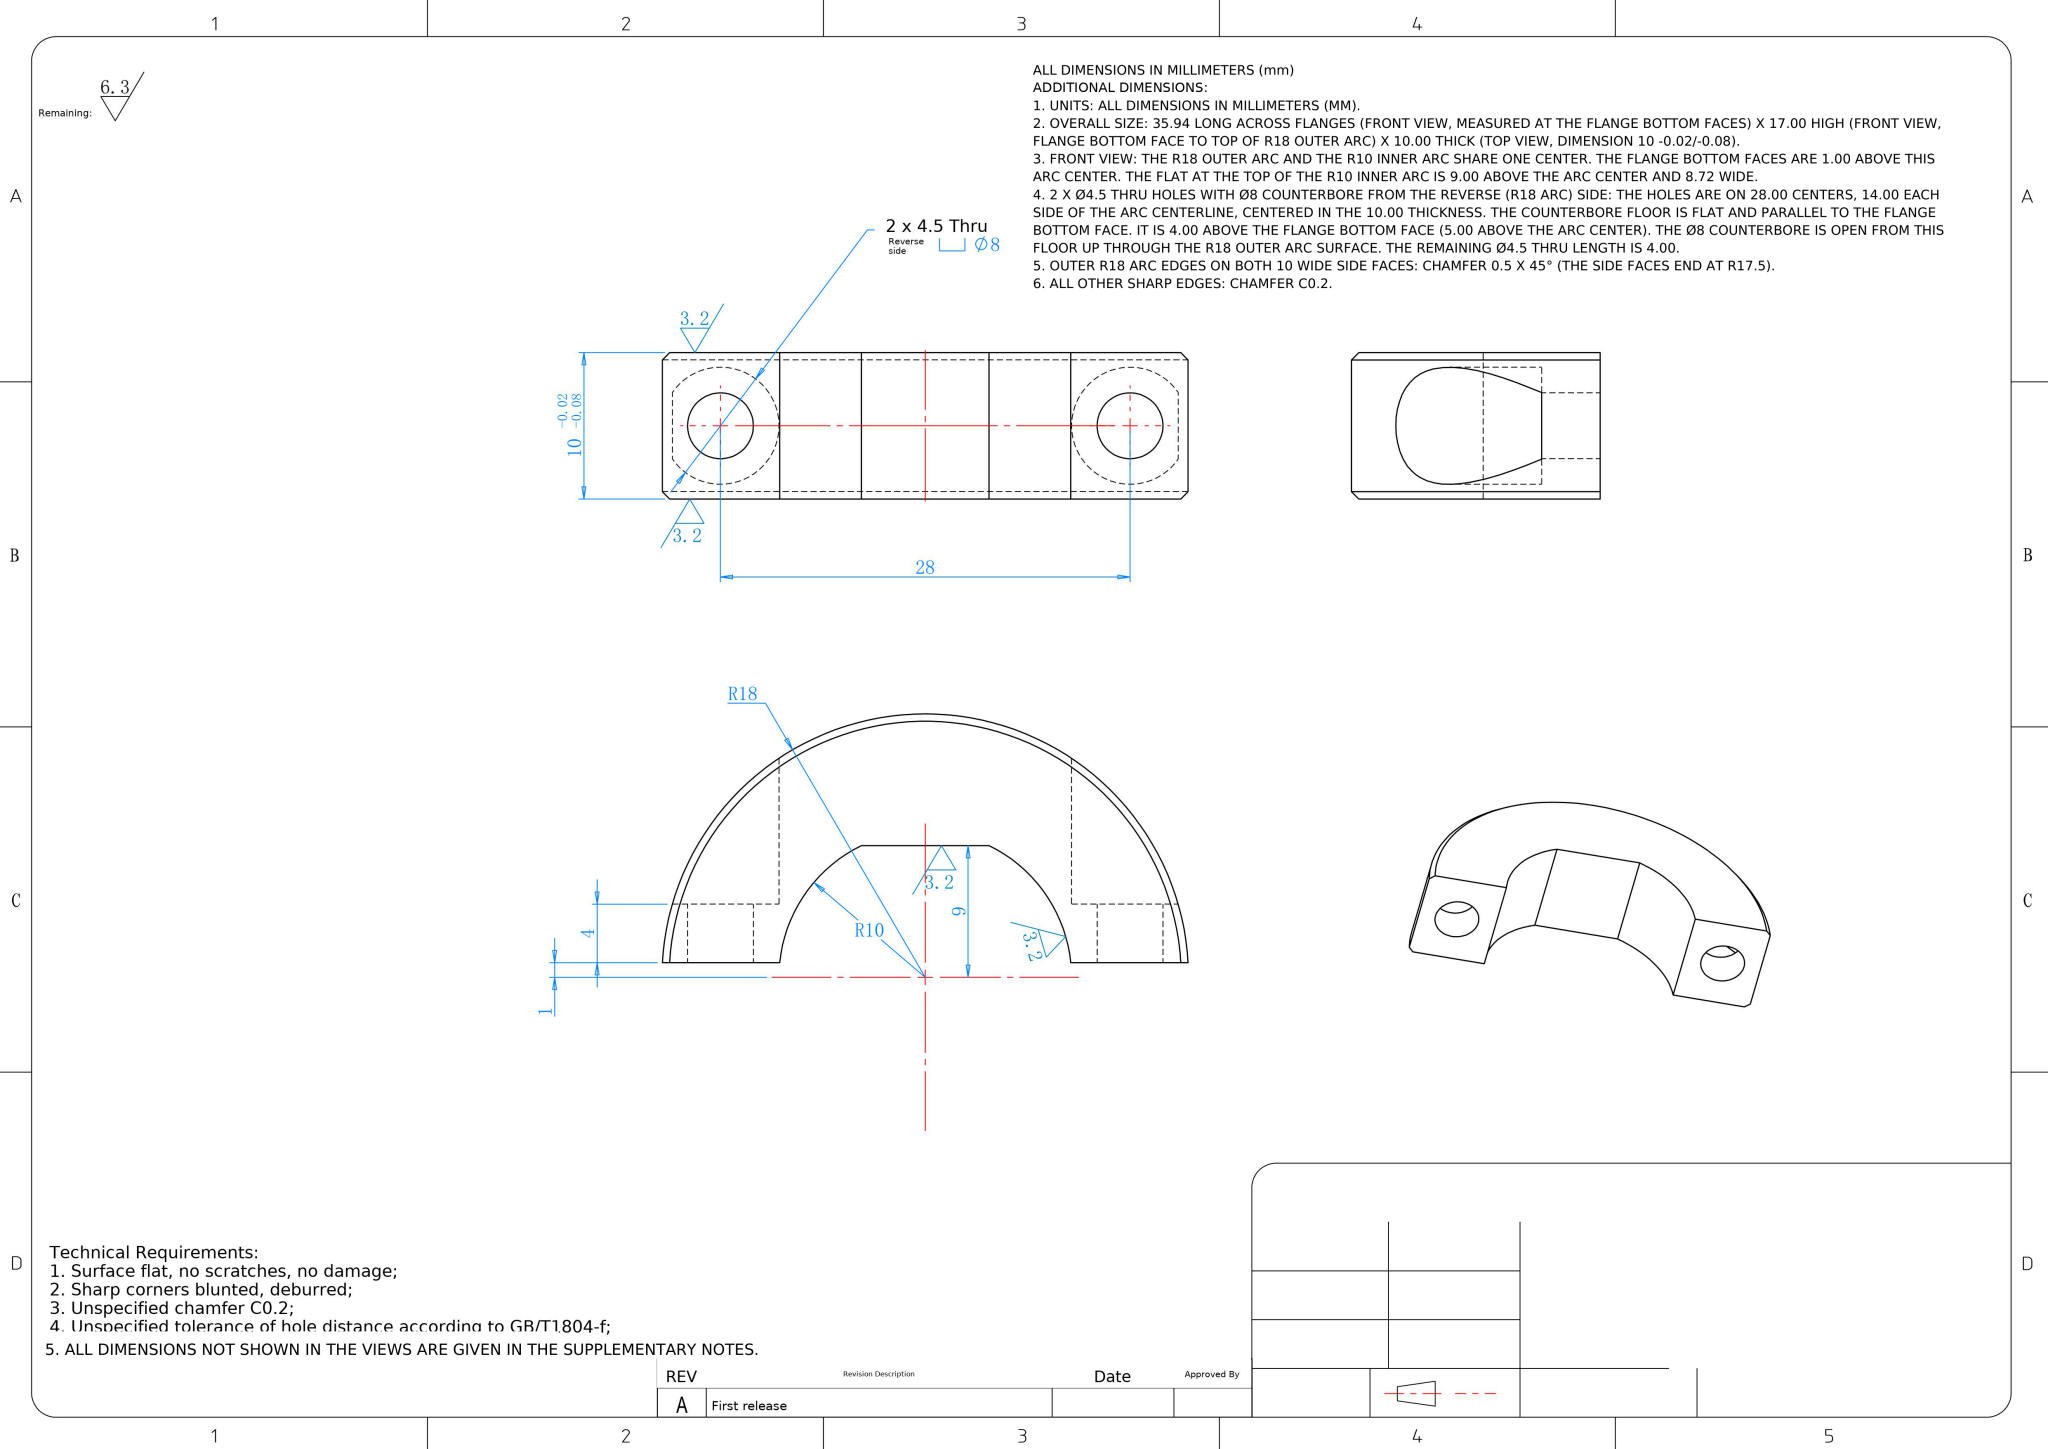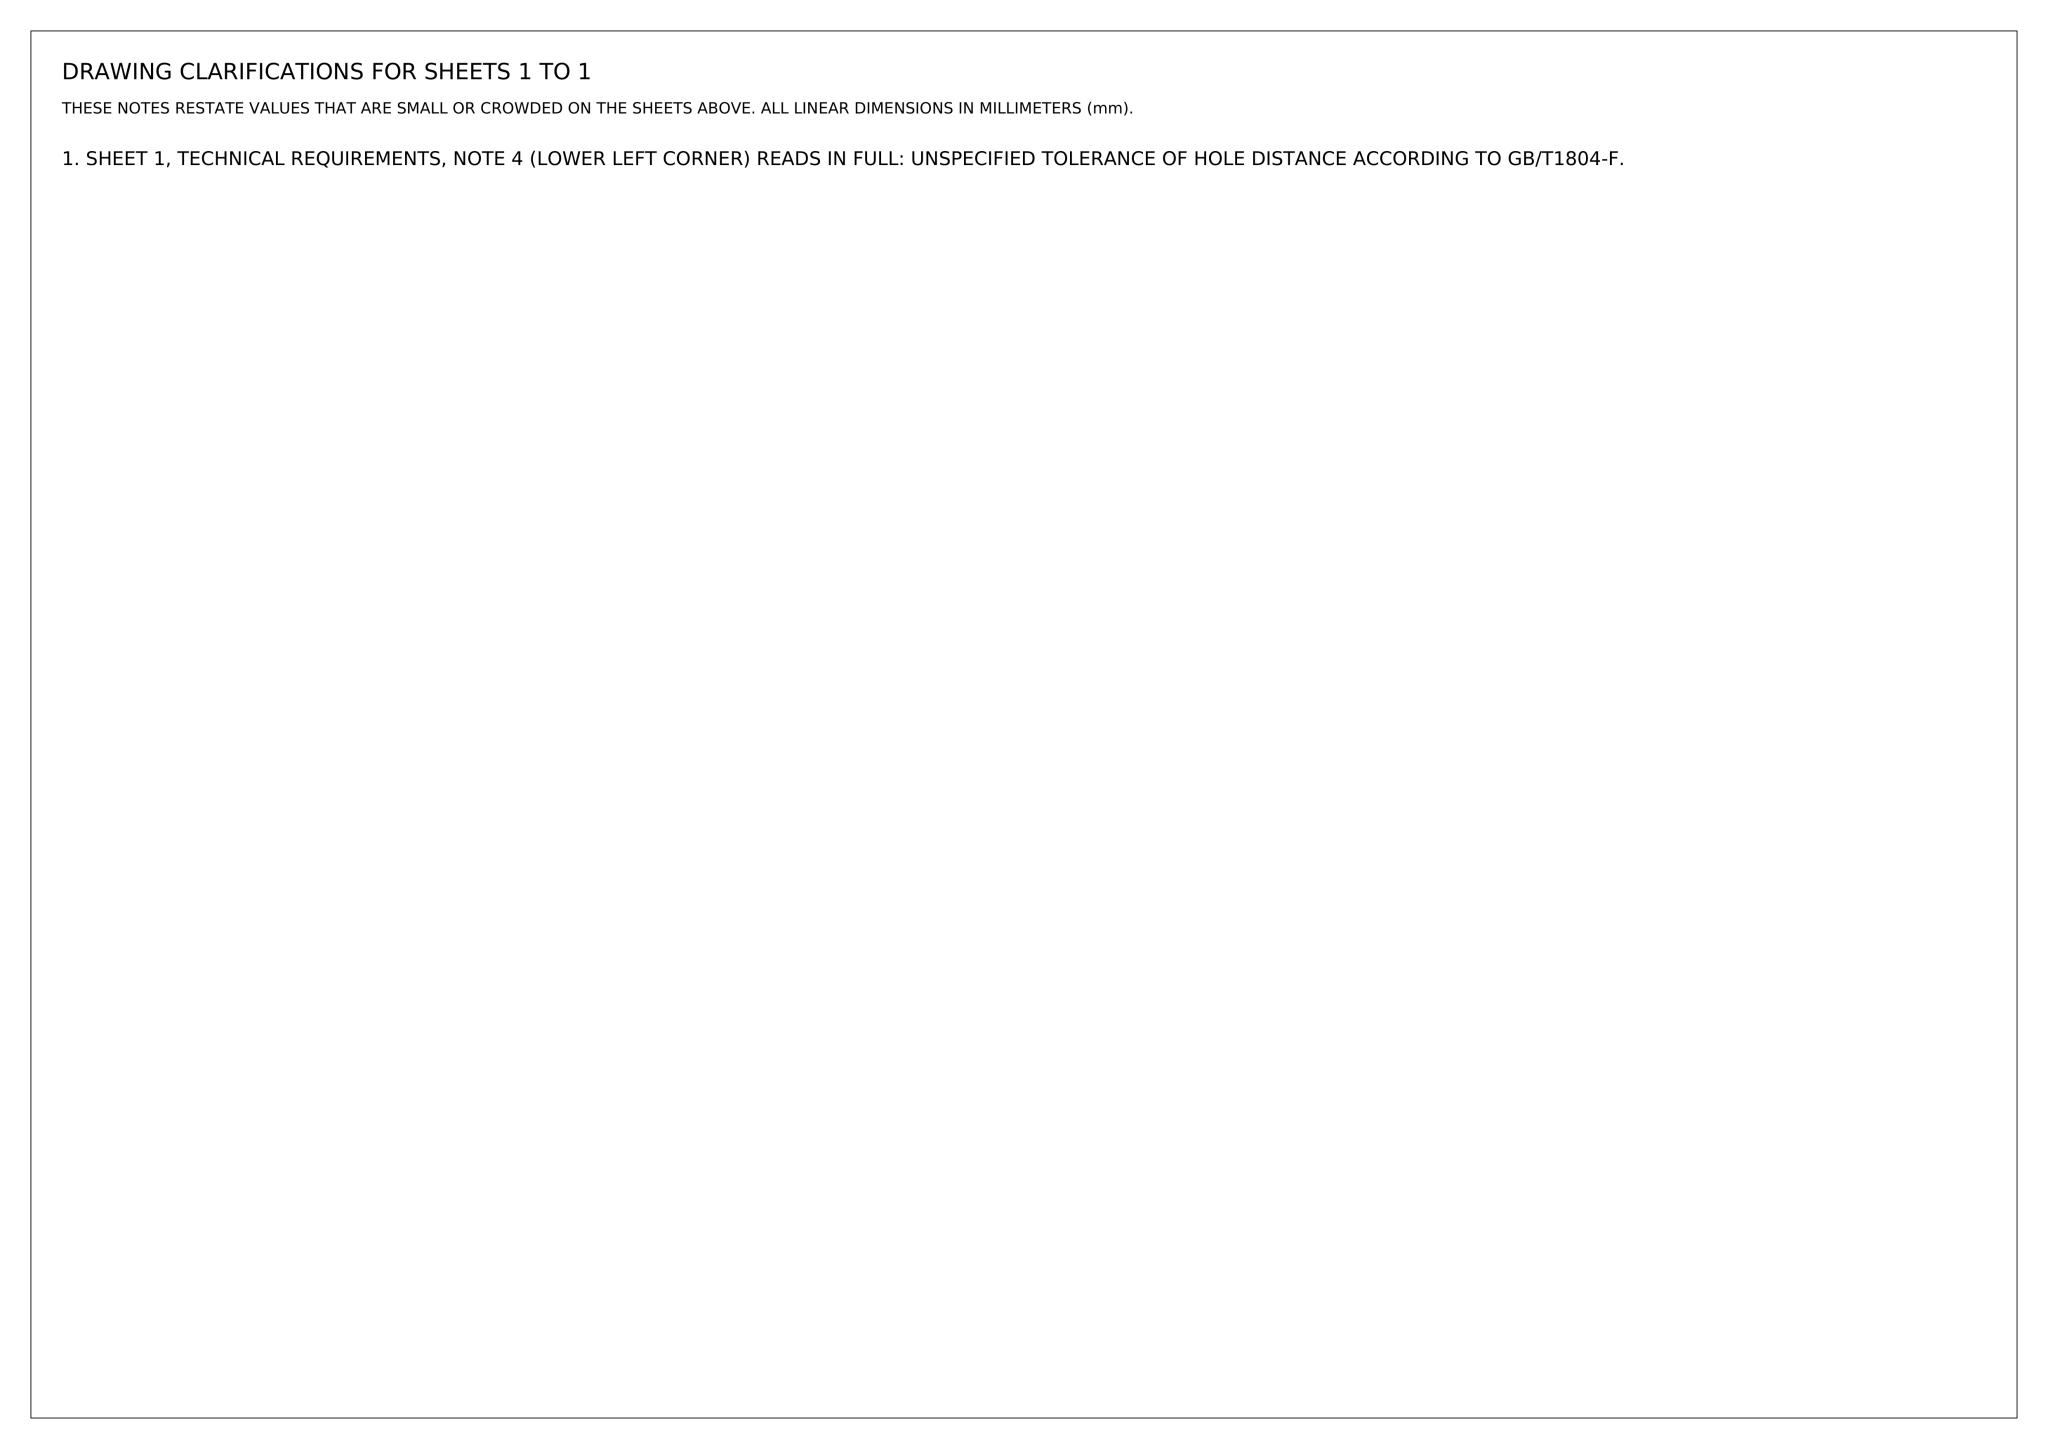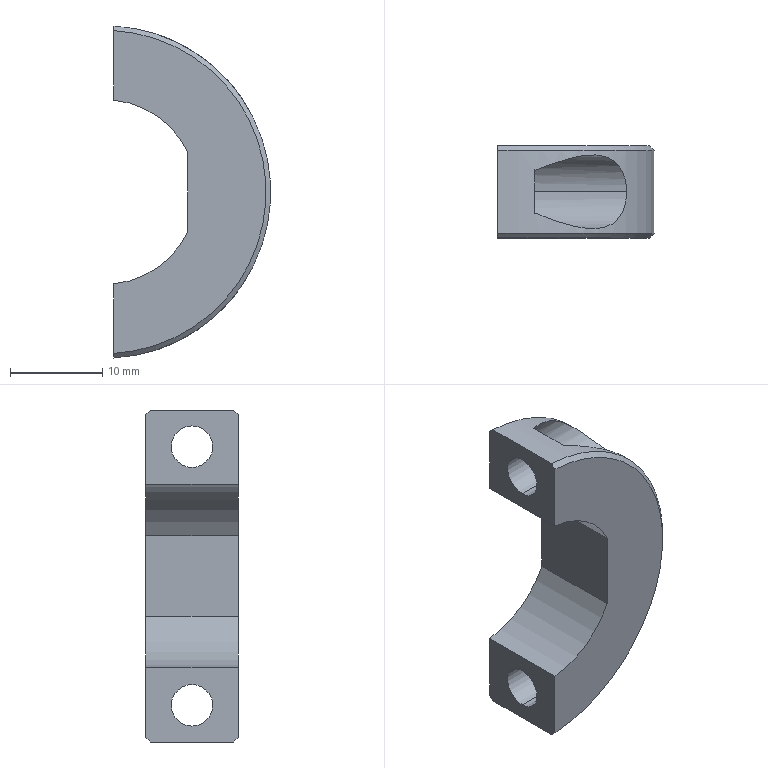Part | NX | mm | 1 solid | 19 faces | box 17 x 10 x 35.94 mm | volume 2692 mm3 | cylinder 10 | plane 7 | cone 2 | commonest cylinder face diameters 4.5 x4 8 x3 20 x2 36 x1
STEP:
#1=COLOUR_RGB('',0.7922,0.8196,0.9333);
#2=FILL_AREA_STYLE_COLOUR('',#1);
#3=FILL_AREA_STYLE('',(#2));
#4=SURFACE_STYLE_FILL_AREA(#3);
#5=SURFACE_SIDE_STYLE('',(#4));
#6=SURFACE_STYLE_USAGE(.BOTH.,#5);
#7=PRESENTATION_STYLE_ASSIGNMENT((#6));
#8=CARTESIAN_POINT('',(1.,0.,16.25));
#9=VERTEX_POINT('',#8);
#10=CARTESIAN_POINT('',(1.,0.,11.75));
#11=VERTEX_POINT('',#10);
#12=CARTESIAN_POINT('',(1.,0.,14.));
#13=DIRECTION('',(1.,0.,0.));
#14=DIRECTION('',(0.,0.,-1.));
#15=AXIS2_PLACEMENT_3D('',#12,#13,#14);
#16=CIRCLE('',#15,2.25);
#17=EDGE_CURVE('',#9,#11,#16,.T.);
#18=ORIENTED_EDGE('',*,*,#17,.F.);
#19=CARTESIAN_POINT('',(5.,0.,16.25));
#20=VERTEX_POINT('',#19);
#21=CARTESIAN_POINT('',(16.,0.,16.25));
#22=DIRECTION('',(1.,0.,0.));
#23=VECTOR('',#22,1000.);
#24=LINE('',#21,#23);
#25=EDGE_CURVE('',#9,#20,#24,.T.);
#26=ORIENTED_EDGE('',*,*,#25,.T.);
#27=CARTESIAN_POINT('',(5.,0.,11.75));
#28=VERTEX_POINT('',#27);
#29=CARTESIAN_POINT('',(5.,0.,14.));
#30=DIRECTION('',(1.,0.,0.));
#31=DIRECTION('',(0.,0.,-1.));
#32=AXIS2_PLACEMENT_3D('',#29,#30,#31);
#33=CIRCLE('',#32,2.25);
#34=EDGE_CURVE('',#20,#28,#33,.T.);
#35=ORIENTED_EDGE('',*,*,#34,.T.);
#36=CARTESIAN_POINT('',(16.,0.,11.75));
#37=DIRECTION('',(1.,0.,0.));
#38=VECTOR('',#37,1000.);
#39=LINE('',#36,#38);
#40=EDGE_CURVE('',#11,#28,#39,.T.);
#41=ORIENTED_EDGE('',*,*,#40,.F.);
#42=EDGE_LOOP('',(#18,#26,#35,#41));
#43=FACE_OUTER_BOUND('',#42,.T.);
#44=CARTESIAN_POINT('',(16.,0.,14.));
#45=DIRECTION('',(1.,0.,0.));
#46=DIRECTION('',(0.,0.,-1.));
#47=AXIS2_PLACEMENT_3D('',#44,#45,#46);
#48=CYLINDRICAL_SURFACE('',#47,2.25);
#49=ADVANCED_FACE('',(#43),#48,.F.);
#50=CARTESIAN_POINT('',(5.,0.,10.));
#51=VERTEX_POINT('',#50);
#52=CARTESIAN_POINT('',(5.,2.273,17.292));
#53=VERTEX_POINT('',#52);
#54=CARTESIAN_POINT('',(5.,0.,14.));
#55=DIRECTION('',(1.,0.,0.));
#56=DIRECTION('',(0.,0.,-1.));
#57=AXIS2_PLACEMENT_3D('',#54,#55,#56);
#58=CIRCLE('',#57,4.);
#59=EDGE_CURVE('',#51,#53,#58,.T.);
#60=ORIENTED_EDGE('',*,*,#59,.F.);
#61=CARTESIAN_POINT('',(14.967,-0.,10.));
#62=VERTEX_POINT('',#61);
#63=CARTESIAN_POINT('',(16.,0.,10.));
#64=DIRECTION('',(1.,0.,0.));
#65=VECTOR('',#64,1000.);
#66=LINE('',#63,#65);
#67=EDGE_CURVE('',#51,#62,#66,.T.);
#68=ORIENTED_EDGE('',*,*,#67,.T.);
#69=CARTESIAN_POINT('',(5.,2.273,17.292));
#70=CARTESIAN_POINT('',(6.112,2.738,16.97));
#71=CARTESIAN_POINT('',(7.192,3.151,16.544));
#72=CARTESIAN_POINT('',(8.78,3.623,15.725));
#73=CARTESIAN_POINT('',(9.304,3.755,15.421));
#74=CARTESIAN_POINT('',(10.343,3.946,14.745));
#75=CARTESIAN_POINT('',(10.844,4.001,14.38));
#76=CARTESIAN_POINT('',(11.571,3.999,13.791));
#77=CARTESIAN_POINT('',(11.811,3.984,13.587));
#78=CARTESIAN_POINT('',(12.273,3.919,13.171));
#79=CARTESIAN_POINT('',(12.495,3.869,12.96));
#80=CARTESIAN_POINT('',(12.924,3.728,12.532));
#81=CARTESIAN_POINT('',(13.13,3.637,12.316));
#82=CARTESIAN_POINT('',(13.523,3.403,11.883));
#83=CARTESIAN_POINT('',(13.706,3.263,11.672));
#84=CARTESIAN_POINT('',(14.042,2.931,11.265));
#85=CARTESIAN_POINT('',(14.197,2.735,11.067));
#86=CARTESIAN_POINT('',(14.467,2.296,10.713));
#87=CARTESIAN_POINT('',(14.582,2.053,10.554));
#88=CARTESIAN_POINT('',(14.773,1.513,10.285));
#89=CARTESIAN_POINT('',(14.844,1.229,10.181));
#90=CARTESIAN_POINT('',(14.917,0.7788,10.074));
#91=CARTESIAN_POINT('',(14.936,0.6238,10.046));
#92=CARTESIAN_POINT('',(14.961,0.3119,10.009));
#93=CARTESIAN_POINT('',(14.967,0.1559,10.));
#94=CARTESIAN_POINT('',(14.967,-0.,10.));
#95=B_SPLINE_CURVE_WITH_KNOTS('',3,(#69,#70,#71,#72,#73,#74,#75,#76,#77,#78,#79,#80,#81,#82,#83,#84,#85,#86,#87,#88,#89,#90,#91,#92,#93,#94),.UNSPECIFIED.,.F.,.F.,(4,2,2,2,2,2,2,2,2,2,2,2,4),(0.,0.00369,0.005535,0.007379,0.008302,0.009224,0.01015,0.01107,0.01199,0.01291,0.01384,0.0143,0.01476),.UNSPECIFIED.);
#96=EDGE_CURVE('',#53,#62,#95,.T.);
#97=ORIENTED_EDGE('',*,*,#96,.F.);
#98=EDGE_LOOP('',(#60,#68,#97));
#99=FACE_OUTER_BOUND('',#98,.T.);
#100=CARTESIAN_POINT('',(16.,0.,14.));
#101=DIRECTION('',(1.,0.,0.));
#102=DIRECTION('',(0.,0.,-1.));
#103=AXIS2_PLACEMENT_3D('',#100,#101,#102);
#104=CYLINDRICAL_SURFACE('',#103,4.);
#105=ADVANCED_FACE('',(#99),#104,.F.);
#106=CARTESIAN_POINT('',(1.,0.,-11.75));
#107=VERTEX_POINT('',#106);
#108=CARTESIAN_POINT('',(1.,0.,-16.25));
#109=VERTEX_POINT('',#108);
#110=CARTESIAN_POINT('',(1.,0.,-14.));
#111=DIRECTION('',(1.,0.,0.));
#112=DIRECTION('',(0.,0.,-1.));
#113=AXIS2_PLACEMENT_3D('',#110,#111,#112);
#114=CIRCLE('',#113,2.25);
#115=EDGE_CURVE('',#107,#109,#114,.T.);
#116=ORIENTED_EDGE('',*,*,#115,.F.);
#117=CARTESIAN_POINT('',(5.,0.,-11.75));
#118=VERTEX_POINT('',#117);
#119=CARTESIAN_POINT('',(16.,0.,-11.75));
#120=DIRECTION('',(1.,0.,0.));
#121=VECTOR('',#120,1000.);
#122=LINE('',#119,#121);
#123=EDGE_CURVE('',#107,#118,#122,.T.);
#124=ORIENTED_EDGE('',*,*,#123,.T.);
#125=CARTESIAN_POINT('',(5.,0.,-16.25));
#126=VERTEX_POINT('',#125);
#127=CARTESIAN_POINT('',(5.,0.,-14.));
#128=DIRECTION('',(1.,0.,0.));
#129=DIRECTION('',(0.,0.,-1.));
#130=AXIS2_PLACEMENT_3D('',#127,#128,#129);
#131=CIRCLE('',#130,2.25);
#132=EDGE_CURVE('',#118,#126,#131,.T.);
#133=ORIENTED_EDGE('',*,*,#132,.T.);
#134=CARTESIAN_POINT('',(16.,0.,-16.25));
#135=DIRECTION('',(1.,0.,0.));
#136=VECTOR('',#135,1000.);
#137=LINE('',#134,#136);
#138=EDGE_CURVE('',#109,#126,#137,.T.);
#139=ORIENTED_EDGE('',*,*,#138,.F.);
#140=EDGE_LOOP('',(#116,#124,#133,#139));
#141=FACE_OUTER_BOUND('',#140,.T.);
#142=CARTESIAN_POINT('',(16.,0.,-14.));
#143=DIRECTION('',(1.,0.,0.));
#144=DIRECTION('',(0.,0.,-1.));
#145=AXIS2_PLACEMENT_3D('',#142,#143,#144);
#146=CYLINDRICAL_SURFACE('',#145,2.25);
#147=ADVANCED_FACE('',(#141),#146,.F.);
#148=CARTESIAN_POINT('',(9.,-5.,-4.359));
#149=VERTEX_POINT('',#148);
#150=CARTESIAN_POINT('',(9.,5.,-4.359));
#151=VERTEX_POINT('',#150);
#152=CARTESIAN_POINT('',(9.,-13.775,-4.359));
#153=DIRECTION('',(0.,1.,0.));
#154=VECTOR('',#153,1000.);
#155=LINE('',#152,#154);
#156=EDGE_CURVE('',#149,#151,#155,.T.);
#157=ORIENTED_EDGE('',*,*,#156,.T.);
#158=CARTESIAN_POINT('',(1.,5.,-9.95));
#159=VERTEX_POINT('',#158);
#160=CARTESIAN_POINT('',(0.,5.,0.));
#161=DIRECTION('',(0.,1.,0.));
#162=DIRECTION('',(0.,0.,1.));
#163=AXIS2_PLACEMENT_3D('',#160,#161,#162);
#164=CIRCLE('',#163,10.);
#165=EDGE_CURVE('',#151,#159,#164,.T.);
#166=ORIENTED_EDGE('',*,*,#165,.T.);
#167=CARTESIAN_POINT('',(1.,-5.,-9.95));
#168=VERTEX_POINT('',#167);
#169=CARTESIAN_POINT('',(1.,5.,-9.95));
#170=DIRECTION('',(0.,1.,0.));
#171=VECTOR('',#170,1000.);
#172=LINE('',#169,#171);
#173=EDGE_CURVE('',#168,#159,#172,.T.);
#174=ORIENTED_EDGE('',*,*,#173,.F.);
#175=CARTESIAN_POINT('',(0.,-5.,0.));
#176=DIRECTION('',(0.,1.,0.));
#177=DIRECTION('',(0.,0.,1.));
#178=AXIS2_PLACEMENT_3D('',#175,#176,#177);
#179=CIRCLE('',#178,10.);
#180=EDGE_CURVE('',#149,#168,#179,.T.);
#181=ORIENTED_EDGE('',*,*,#180,.F.);
#182=EDGE_LOOP('',(#157,#166,#174,#181));
#183=FACE_OUTER_BOUND('',#182,.T.);
#184=CARTESIAN_POINT('',(0.,5.,0.));
#185=DIRECTION('',(0.,-1.,0.));
#186=DIRECTION('',(0.,0.,-1.));
#187=AXIS2_PLACEMENT_3D('',#184,#185,#186);
#188=CYLINDRICAL_SURFACE('',#187,10.);
#189=ADVANCED_FACE('',(#183),#188,.F.);
#190=CARTESIAN_POINT('',(1.,5.,17.471));
#191=VERTEX_POINT('',#190);
#192=CARTESIAN_POINT('',(1.,5.,9.95));
#193=VERTEX_POINT('',#192);
#194=CARTESIAN_POINT('',(1.,5.,-25.));
#195=DIRECTION('',(-0.,0.,-1.));
#196=VECTOR('',#195,1000.);
#197=LINE('',#194,#196);
#198=EDGE_CURVE('',#191,#193,#197,.T.);
#199=ORIENTED_EDGE('',*,*,#198,.F.);
#200=CARTESIAN_POINT('',(1.,5.,-17.471));
#201=VERTEX_POINT('',#200);
#202=CARTESIAN_POINT('',(0.,5.,0.));
#203=DIRECTION('',(0.,1.,0.));
#204=DIRECTION('',(0.,0.,1.));
#205=AXIS2_PLACEMENT_3D('',#202,#203,#204);
#206=CIRCLE('',#205,17.5);
#207=EDGE_CURVE('',#191,#201,#206,.T.);
#208=ORIENTED_EDGE('',*,*,#207,.T.);
#209=CARTESIAN_POINT('',(1.,5.,-25.));
#210=DIRECTION('',(-0.,0.,-1.));
#211=VECTOR('',#210,1000.);
#212=LINE('',#209,#211);
#213=EDGE_CURVE('',#159,#201,#212,.T.);
#214=ORIENTED_EDGE('',*,*,#213,.F.);
#215=ORIENTED_EDGE('',*,*,#165,.F.);
#216=CARTESIAN_POINT('',(9.,5.,4.359));
#217=VERTEX_POINT('',#216);
#218=CARTESIAN_POINT('',(9.,5.,-4.359));
#219=DIRECTION('',(0.,0.,1.));
#220=VECTOR('',#219,1000.);
#221=LINE('',#218,#220);
#222=EDGE_CURVE('',#151,#217,#221,.T.);
#223=ORIENTED_EDGE('',*,*,#222,.T.);
#224=CARTESIAN_POINT('',(0.,5.,0.));
#225=DIRECTION('',(0.,1.,0.));
#226=DIRECTION('',(0.,0.,1.));
#227=AXIS2_PLACEMENT_3D('',#224,#225,#226);
#228=CIRCLE('',#227,10.);
#229=EDGE_CURVE('',#193,#217,#228,.T.);
#230=ORIENTED_EDGE('',*,*,#229,.F.);
#231=EDGE_LOOP('',(#199,#208,#214,#215,#223,#230));
#232=FACE_OUTER_BOUND('',#231,.T.);
#233=CARTESIAN_POINT('',(0.,5.,0.));
#234=DIRECTION('',(0.,1.,0.));
#235=DIRECTION('',(0.,0.,1.));
#236=AXIS2_PLACEMENT_3D('',#233,#234,#235);
#237=PLANE('',#236);
#238=ADVANCED_FACE('',(#232),#237,.T.);
#239=CARTESIAN_POINT('',(1.,-5.,-17.471));
#240=VERTEX_POINT('',#239);
#241=CARTESIAN_POINT('',(1.,-5.,-25.));
#242=DIRECTION('',(-0.,0.,-1.));
#243=VECTOR('',#242,1000.);
#244=LINE('',#241,#243);
#245=EDGE_CURVE('',#168,#240,#244,.T.);
#246=ORIENTED_EDGE('',*,*,#245,.T.);
#247=CARTESIAN_POINT('',(1.,-5.,17.471));
#248=VERTEX_POINT('',#247);
#249=CARTESIAN_POINT('',(0.,-5.,0.));
#250=DIRECTION('',(0.,-1.,0.));
#251=DIRECTION('',(0.,0.,1.));
#252=AXIS2_PLACEMENT_3D('',#249,#250,#251);
#253=CIRCLE('',#252,17.5);
#254=EDGE_CURVE('',#240,#248,#253,.T.);
#255=ORIENTED_EDGE('',*,*,#254,.T.);
#256=CARTESIAN_POINT('',(1.,-5.,9.95));
#257=VERTEX_POINT('',#256);
#258=CARTESIAN_POINT('',(1.,-5.,-25.));
#259=DIRECTION('',(-0.,0.,-1.));
#260=VECTOR('',#259,1000.);
#261=LINE('',#258,#260);
#262=EDGE_CURVE('',#248,#257,#261,.T.);
#263=ORIENTED_EDGE('',*,*,#262,.T.);
#264=CARTESIAN_POINT('',(9.,-5.,4.359));
#265=VERTEX_POINT('',#264);
#266=CARTESIAN_POINT('',(0.,-5.,0.));
#267=DIRECTION('',(0.,1.,0.));
#268=DIRECTION('',(0.,0.,1.));
#269=AXIS2_PLACEMENT_3D('',#266,#267,#268);
#270=CIRCLE('',#269,10.);
#271=EDGE_CURVE('',#257,#265,#270,.T.);
#272=ORIENTED_EDGE('',*,*,#271,.T.);
#273=CARTESIAN_POINT('',(9.,-5.,-4.359));
#274=DIRECTION('',(0.,0.,-1.));
#275=VECTOR('',#274,1000.);
#276=LINE('',#273,#275);
#277=EDGE_CURVE('',#265,#149,#276,.T.);
#278=ORIENTED_EDGE('',*,*,#277,.T.);
#279=ORIENTED_EDGE('',*,*,#180,.T.);
#280=EDGE_LOOP('',(#246,#255,#263,#272,#278,#279));
#281=FACE_OUTER_BOUND('',#280,.T.);
#282=CARTESIAN_POINT('',(0.,-5.,0.));
#283=DIRECTION('',(0.,1.,0.));
#284=DIRECTION('',(0.,0.,1.));
#285=AXIS2_PLACEMENT_3D('',#282,#283,#284);
#286=PLANE('',#285);
#287=ADVANCED_FACE('',(#281),#286,.F.);
#288=ORIENTED_EDGE('',*,*,#96,.T.);
#289=CARTESIAN_POINT('',(5.,-2.273,17.292));
#290=VERTEX_POINT('',#289);
#291=CARTESIAN_POINT('',(14.967,-0.,10.));
#292=CARTESIAN_POINT('',(14.967,-0.1555,10.));
#293=CARTESIAN_POINT('',(14.961,-0.311,10.009));
#294=CARTESIAN_POINT('',(14.936,-0.622,10.046));
#295=CARTESIAN_POINT('',(14.918,-0.7768,10.073));
#296=CARTESIAN_POINT('',(14.869,-1.077,10.145));
#297=CARTESIAN_POINT('',(14.839,-1.223,10.189));
#298=CARTESIAN_POINT('',(14.767,-1.509,10.292));
#299=CARTESIAN_POINT('',(14.725,-1.649,10.353));
#300=CARTESIAN_POINT('',(14.583,-2.051,10.553));
#301=CARTESIAN_POINT('',(14.468,-2.294,10.711));
#302=CARTESIAN_POINT('',(14.197,-2.736,11.068));
#303=CARTESIAN_POINT('',(14.044,-2.928,11.263));
#304=CARTESIAN_POINT('',(13.707,-3.262,11.67));
#305=CARTESIAN_POINT('',(13.522,-3.404,11.885));
#306=CARTESIAN_POINT('',(13.133,-3.635,12.312));
#307=CARTESIAN_POINT('',(12.929,-3.726,12.527));
#308=CARTESIAN_POINT('',(12.499,-3.868,12.956));
#309=CARTESIAN_POINT('',(12.273,-3.919,13.17));
#310=CARTESIAN_POINT('',(11.814,-3.984,13.584));
#311=CARTESIAN_POINT('',(11.578,-3.999,13.785));
#312=CARTESIAN_POINT('',(11.098,-4.001,14.175));
#313=CARTESIAN_POINT('',(10.852,-3.988,14.364));
#314=CARTESIAN_POINT('',(10.35,-3.937,14.73));
#315=CARTESIAN_POINT('',(10.094,-3.9,14.907));
#316=CARTESIAN_POINT('',(9.322,-3.759,15.41));
#317=CARTESIAN_POINT('',(8.801,-3.628,15.713));
#318=CARTESIAN_POINT('',(7.741,-3.314,16.262));
#319=CARTESIAN_POINT('',(7.202,-3.131,16.507));
#320=CARTESIAN_POINT('',(6.107,-2.726,16.943));
#321=CARTESIAN_POINT('',(5.556,-2.505,17.131));
#322=CARTESIAN_POINT('',(5.,-2.273,17.292));
#323=B_SPLINE_CURVE_WITH_KNOTS('',3,(#291,#292,#293,#294,#295,#296,#297,#298,#299,#300,#301,#302,#303,#304,#305,#306,#307,#308,#309,#310,#311,#312,#313,#314,#315,#316,#317,#318,#319,#320,#321,#322),.UNSPECIFIED.,.F.,.F.,(4,2,2,2,2,2,2,2,2,2,2,2,2,2,2,4),(0.01476,0.01522,0.01568,0.01614,0.0166,0.01752,0.01844,0.01936,0.02028,0.0212,0.02212,0.02304,0.02396,0.0258,0.02764,0.02948),.UNSPECIFIED.);
#324=EDGE_CURVE('',#62,#290,#323,.T.);
#325=ORIENTED_EDGE('',*,*,#324,.T.);
#326=CARTESIAN_POINT('',(5.,5.,17.292));
#327=DIRECTION('',(0.,1.,0.));
#328=VECTOR('',#327,1000.);
#329=LINE('',#326,#328);
#330=EDGE_CURVE('',#290,#53,#329,.T.);
#331=ORIENTED_EDGE('',*,*,#330,.T.);
#332=EDGE_LOOP('',(#288,#325,#331));
#333=FACE_BOUND('',#332,.T.);
#334=CARTESIAN_POINT('',(5.,-2.273,-17.292));
#335=VERTEX_POINT('',#334);
#336=CARTESIAN_POINT('',(5.,2.273,-17.292));
#337=VERTEX_POINT('',#336);
#338=CARTESIAN_POINT('',(5.,-2.273,-17.292));
#339=CARTESIAN_POINT('',(6.11,-2.738,-16.971));
#340=CARTESIAN_POINT('',(7.19,-3.15,-16.545));
#341=CARTESIAN_POINT('',(8.775,-3.621,-15.727));
#342=CARTESIAN_POINT('',(9.298,-3.754,-15.425));
#343=CARTESIAN_POINT('',(10.336,-3.945,-14.75));
#344=CARTESIAN_POINT('',(10.837,-4.001,-14.386));
#345=CARTESIAN_POINT('',(11.563,-4.,-13.798));
#346=CARTESIAN_POINT('',(11.802,-3.985,-13.594));
#347=CARTESIAN_POINT('',(12.264,-3.92,-13.179));
#348=CARTESIAN_POINT('',(12.487,-3.871,-12.968));
#349=CARTESIAN_POINT('',(12.915,-3.731,-12.541));
#350=CARTESIAN_POINT('',(13.122,-3.641,-12.325));
#351=CARTESIAN_POINT('',(13.515,-3.409,-11.892));
#352=CARTESIAN_POINT('',(13.697,-3.27,-11.681));
#353=CARTESIAN_POINT('',(14.034,-2.939,-11.275));
#354=CARTESIAN_POINT('',(14.19,-2.745,-11.077));
#355=CARTESIAN_POINT('',(14.46,-2.309,-10.721));
#356=CARTESIAN_POINT('',(14.576,-2.067,-10.562));
#357=CARTESIAN_POINT('',(14.769,-1.529,-10.292));
#358=CARTESIAN_POINT('',(14.841,-1.245,-10.186));
#359=CARTESIAN_POINT('',(14.94,-0.6477,-10.041));
#360=CARTESIAN_POINT('',(14.966,-0.3312,-10.002));
#361=CARTESIAN_POINT('',(14.967,0.1359,-9.999));
#362=CARTESIAN_POINT('',(14.962,0.2917,-10.008));
#363=CARTESIAN_POINT('',(14.938,0.6031,-10.043));
#364=CARTESIAN_POINT('',(14.92,0.7584,-10.07));
#365=CARTESIAN_POINT('',(14.872,1.059,-10.14));
#366=CARTESIAN_POINT('',(14.843,1.206,-10.183));
#367=CARTESIAN_POINT('',(14.772,1.493,-10.286));
#368=CARTESIAN_POINT('',(14.73,1.634,-10.346));
#369=CARTESIAN_POINT('',(14.589,2.037,-10.545));
#370=CARTESIAN_POINT('',(14.474,2.282,-10.702));
#371=CARTESIAN_POINT('',(14.204,2.726,-11.059));
#372=CARTESIAN_POINT('',(14.051,2.919,-11.253));
#373=CARTESIAN_POINT('',(13.715,3.255,-11.66));
#374=CARTESIAN_POINT('',(13.53,3.398,-11.875));
#375=CARTESIAN_POINT('',(13.142,3.631,-12.303));
#376=CARTESIAN_POINT('',(12.938,3.722,-12.519));
#377=CARTESIAN_POINT('',(12.508,3.866,-12.948));
#378=CARTESIAN_POINT('',(12.282,3.917,-13.163));
#379=CARTESIAN_POINT('',(11.822,3.983,-13.577));
#380=CARTESIAN_POINT('',(11.586,3.999,-13.779));
#381=CARTESIAN_POINT('',(11.105,4.001,-14.169));
#382=CARTESIAN_POINT('',(10.859,3.988,-14.359));
#383=CARTESIAN_POINT('',(10.357,3.938,-14.725));
#384=CARTESIAN_POINT('',(10.1,3.901,-14.902));
#385=CARTESIAN_POINT('',(9.328,3.761,-15.407));
#386=CARTESIAN_POINT('',(8.806,3.63,-15.71));
#387=CARTESIAN_POINT('',(7.744,3.316,-16.26));
#388=CARTESIAN_POINT('',(7.205,3.132,-16.506));
#389=CARTESIAN_POINT('',(6.108,2.726,-16.942));
#390=CARTESIAN_POINT('',(5.556,2.506,-17.131));
#391=CARTESIAN_POINT('',(5.,2.273,-17.292));
#392=B_SPLINE_CURVE_WITH_KNOTS('',3,(#338,#339,#340,#341,#342,#343,#344,#345,#346,#347,#348,#349,#350,#351,#352,#353,#354,#355,#356,#357,#358,#359,#360,#361,#362,#363,#364,#365,#366,#367,#368,#369,#370,#371,#372,#373,#374,#375,#376,#377,#378,#379,#380,#381,#382,#383,#384,#385,#386,#387,#388,#389,#390,#391),.UNSPECIFIED.,.F.,.F.,(4,2,2,2,2,2,2,2,2,2,2,2,2,2,2,2,2,2,2,2,2,2,2,2,2,2,4),(0.,0.003685,0.005527,0.00737,0.008291,0.009212,0.01013,0.01105,0.01198,0.0129,0.01382,0.01474,0.0152,0.01566,0.01612,0.01658,0.0175,0.01842,0.01935,0.02027,0.02119,0.02211,0.02303,0.02395,0.02579,0.02764,0.02948),.UNSPECIFIED.);
#393=EDGE_CURVE('',#335,#337,#392,.T.);
#394=ORIENTED_EDGE('',*,*,#393,.T.);
#395=CARTESIAN_POINT('',(5.,5.,-17.292));
#396=DIRECTION('',(0.,-1.,0.));
#397=VECTOR('',#396,1000.);
#398=LINE('',#395,#397);
#399=EDGE_CURVE('',#337,#335,#398,.T.);
#400=ORIENTED_EDGE('',*,*,#399,.T.);
#401=EDGE_LOOP('',(#394,#400));
#402=FACE_BOUND('',#401,.T.);
#403=CARTESIAN_POINT('',(1.,4.5,17.972));
#404=VERTEX_POINT('',#403);
#405=CARTESIAN_POINT('',(1.,-4.5,17.972));
#406=VERTEX_POINT('',#405);
#407=CARTESIAN_POINT('',(1.,5.,17.972));
#408=DIRECTION('',(0.,-1.,0.));
#409=VECTOR('',#408,1000.);
#410=LINE('',#407,#409);
#411=EDGE_CURVE('',#404,#406,#410,.T.);
#412=ORIENTED_EDGE('',*,*,#411,.T.);
#413=CARTESIAN_POINT('',(1.,-4.5,-17.972));
#414=VERTEX_POINT('',#413);
#415=CARTESIAN_POINT('',(0.,-4.5,0.));
#416=DIRECTION('',(0.,1.,0.));
#417=DIRECTION('',(0.,0.,1.));
#418=AXIS2_PLACEMENT_3D('',#415,#416,#417);
#419=CIRCLE('',#418,18.);
#420=EDGE_CURVE('',#406,#414,#419,.T.);
#421=ORIENTED_EDGE('',*,*,#420,.T.);
#422=CARTESIAN_POINT('',(1.,4.5,-17.972));
#423=VERTEX_POINT('',#422);
#424=CARTESIAN_POINT('',(1.,5.,-17.972));
#425=DIRECTION('',(0.,1.,0.));
#426=VECTOR('',#425,1000.);
#427=LINE('',#424,#426);
#428=EDGE_CURVE('',#414,#423,#427,.T.);
#429=ORIENTED_EDGE('',*,*,#428,.T.);
#430=CARTESIAN_POINT('',(0.,4.5,0.));
#431=DIRECTION('',(0.,-1.,0.));
#432=DIRECTION('',(0.,0.,1.));
#433=AXIS2_PLACEMENT_3D('',#430,#431,#432);
#434=CIRCLE('',#433,18.);
#435=EDGE_CURVE('',#423,#404,#434,.T.);
#436=ORIENTED_EDGE('',*,*,#435,.T.);
#437=EDGE_LOOP('',(#412,#421,#429,#436));
#438=FACE_OUTER_BOUND('',#437,.T.);
#439=CARTESIAN_POINT('',(0.,5.,0.));
#440=DIRECTION('',(0.,-1.,0.));
#441=DIRECTION('',(0.,0.,-1.));
#442=AXIS2_PLACEMENT_3D('',#439,#440,#441);
#443=CYLINDRICAL_SURFACE('',#442,18.);
#444=ADVANCED_FACE('',(#333,#402,#438),#443,.T.);
#445=CARTESIAN_POINT('',(9.,-13.775,4.359));
#446=DIRECTION('',(0.,1.,0.));
#447=VECTOR('',#446,1000.);
#448=LINE('',#445,#447);
#449=EDGE_CURVE('',#265,#217,#448,.T.);
#450=ORIENTED_EDGE('',*,*,#449,.F.);
#451=ORIENTED_EDGE('',*,*,#271,.F.);
#452=CARTESIAN_POINT('',(1.,5.,9.95));
#453=DIRECTION('',(0.,-1.,0.));
#454=VECTOR('',#453,1000.);
#455=LINE('',#452,#454);
#456=EDGE_CURVE('',#193,#257,#455,.T.);
#457=ORIENTED_EDGE('',*,*,#456,.F.);
#458=ORIENTED_EDGE('',*,*,#229,.T.);
#459=EDGE_LOOP('',(#450,#451,#457,#458));
#460=FACE_OUTER_BOUND('',#459,.T.);
#461=CARTESIAN_POINT('',(0.,5.,0.));
#462=DIRECTION('',(0.,-1.,0.));
#463=DIRECTION('',(0.,0.,-1.));
#464=AXIS2_PLACEMENT_3D('',#461,#462,#463);
#465=CYLINDRICAL_SURFACE('',#464,10.);
#466=ADVANCED_FACE('',(#460),#465,.F.);
#467=CARTESIAN_POINT('',(1.,0.,-14.));
#468=DIRECTION('',(1.,0.,0.));
#469=DIRECTION('',(0.,0.,-1.));
#470=AXIS2_PLACEMENT_3D('',#467,#468,#469);
#471=CIRCLE('',#470,2.25);
#472=EDGE_CURVE('',#109,#107,#471,.T.);
#473=ORIENTED_EDGE('',*,*,#472,.T.);
#474=ORIENTED_EDGE('',*,*,#115,.T.);
#475=EDGE_LOOP('',(#473,#474));
#476=FACE_BOUND('',#475,.T.);
#477=ORIENTED_EDGE('',*,*,#428,.F.);
#478=CARTESIAN_POINT('',(1.,-4.5,-17.972));
#479=CARTESIAN_POINT('',(1.,-4.667,-17.805));
#480=CARTESIAN_POINT('',(1.,-4.833,-17.638));
#481=CARTESIAN_POINT('',(1.,-5.,-17.471));
#482=B_SPLINE_CURVE_WITH_KNOTS('',3,(#478,#479,#480,#481),.UNSPECIFIED.,.F.,.F.,(4,4),(0.,0.0007077),.UNSPECIFIED.);
#483=EDGE_CURVE('',#414,#240,#482,.T.);
#484=ORIENTED_EDGE('',*,*,#483,.T.);
#485=ORIENTED_EDGE('',*,*,#245,.F.);
#486=ORIENTED_EDGE('',*,*,#173,.T.);
#487=ORIENTED_EDGE('',*,*,#213,.T.);
#488=CARTESIAN_POINT('',(1.,5.,-17.471));
#489=CARTESIAN_POINT('',(1.,4.833,-17.638));
#490=CARTESIAN_POINT('',(1.,4.667,-17.805));
#491=CARTESIAN_POINT('',(1.,4.5,-17.972));
#492=B_SPLINE_CURVE_WITH_KNOTS('',3,(#488,#489,#490,#491),.UNSPECIFIED.,.F.,.F.,(4,4),(0.,0.0007077),.UNSPECIFIED.);
#493=EDGE_CURVE('',#201,#423,#492,.T.);
#494=ORIENTED_EDGE('',*,*,#493,.T.);
#495=EDGE_LOOP('',(#477,#484,#485,#486,#487,#494));
#496=FACE_OUTER_BOUND('',#495,.T.);
#497=CARTESIAN_POINT('',(1.,-5.,-25.));
#498=DIRECTION('',(1.,0.,-0.));
#499=DIRECTION('',(-0.,0.,-1.));
#500=AXIS2_PLACEMENT_3D('',#497,#498,#499);
#501=PLANE('',#500);
#502=ADVANCED_FACE('',(#476,#496),#501,.F.);
#503=CARTESIAN_POINT('',(1.,0.,14.));
#504=DIRECTION('',(1.,0.,0.));
#505=DIRECTION('',(0.,0.,-1.));
#506=AXIS2_PLACEMENT_3D('',#503,#504,#505);
#507=CIRCLE('',#506,2.25);
#508=EDGE_CURVE('',#11,#9,#507,.T.);
#509=ORIENTED_EDGE('',*,*,#508,.T.);
#510=ORIENTED_EDGE('',*,*,#17,.T.);
#511=EDGE_LOOP('',(#509,#510));
#512=FACE_BOUND('',#511,.T.);
#513=ORIENTED_EDGE('',*,*,#262,.F.);
#514=CARTESIAN_POINT('',(1.,-5.,17.471));
#515=CARTESIAN_POINT('',(1.,-4.833,17.638));
#516=CARTESIAN_POINT('',(1.,-4.667,17.805));
#517=CARTESIAN_POINT('',(1.,-4.5,17.972));
#518=B_SPLINE_CURVE_WITH_KNOTS('',3,(#514,#515,#516,#517),.UNSPECIFIED.,.F.,.F.,(4,4),(0.,0.0007077),.UNSPECIFIED.);
#519=EDGE_CURVE('',#248,#406,#518,.T.);
#520=ORIENTED_EDGE('',*,*,#519,.T.);
#521=ORIENTED_EDGE('',*,*,#411,.F.);
#522=CARTESIAN_POINT('',(1.,4.5,17.972));
#523=CARTESIAN_POINT('',(1.,4.667,17.805));
#524=CARTESIAN_POINT('',(1.,4.833,17.638));
#525=CARTESIAN_POINT('',(1.,5.,17.471));
#526=B_SPLINE_CURVE_WITH_KNOTS('',3,(#522,#523,#524,#525),.UNSPECIFIED.,.F.,.F.,(4,4),(0.,0.0007077),.UNSPECIFIED.);
#527=EDGE_CURVE('',#404,#191,#526,.T.);
#528=ORIENTED_EDGE('',*,*,#527,.T.);
#529=ORIENTED_EDGE('',*,*,#198,.T.);
#530=ORIENTED_EDGE('',*,*,#456,.T.);
#531=EDGE_LOOP('',(#513,#520,#521,#528,#529,#530));
#532=FACE_OUTER_BOUND('',#531,.T.);
#533=CARTESIAN_POINT('',(1.,-5.,-25.));
#534=DIRECTION('',(1.,0.,-0.));
#535=DIRECTION('',(-0.,0.,-1.));
#536=AXIS2_PLACEMENT_3D('',#533,#534,#535);
#537=PLANE('',#536);
#538=ADVANCED_FACE('',(#512,#532),#537,.F.);
#539=CARTESIAN_POINT('',(5.,0.,-14.));
#540=DIRECTION('',(1.,0.,0.));
#541=DIRECTION('',(0.,0.,-1.));
#542=AXIS2_PLACEMENT_3D('',#539,#540,#541);
#543=CIRCLE('',#542,2.25);
#544=EDGE_CURVE('',#126,#118,#543,.T.);
#545=ORIENTED_EDGE('',*,*,#544,.F.);
#546=ORIENTED_EDGE('',*,*,#132,.F.);
#547=EDGE_LOOP('',(#545,#546));
#548=FACE_BOUND('',#547,.T.);
#549=CARTESIAN_POINT('',(5.,0.,-14.));
#550=DIRECTION('',(1.,0.,0.));
#551=DIRECTION('',(0.,0.,-1.));
#552=AXIS2_PLACEMENT_3D('',#549,#550,#551);
#553=CIRCLE('',#552,4.);
#554=EDGE_CURVE('',#337,#335,#553,.T.);
#555=ORIENTED_EDGE('',*,*,#554,.T.);
#556=ORIENTED_EDGE('',*,*,#399,.F.);
#557=EDGE_LOOP('',(#555,#556));
#558=FACE_OUTER_BOUND('',#557,.T.);
#559=CARTESIAN_POINT('',(5.,2.25,-14.));
#560=DIRECTION('',(-1.,0.,0.));
#561=DIRECTION('',(0.,0.,1.));
#562=AXIS2_PLACEMENT_3D('',#559,#560,#561);
#563=PLANE('',#562);
#564=ADVANCED_FACE('',(#548,#558),#563,.F.);
#565=ORIENTED_EDGE('',*,*,#554,.F.);
#566=ORIENTED_EDGE('',*,*,#393,.F.);
#567=EDGE_LOOP('',(#565,#566));
#568=FACE_OUTER_BOUND('',#567,.T.);
#569=CARTESIAN_POINT('',(16.,0.,-14.));
#570=DIRECTION('',(1.,0.,0.));
#571=DIRECTION('',(0.,0.,-1.));
#572=AXIS2_PLACEMENT_3D('',#569,#570,#571);
#573=CYLINDRICAL_SURFACE('',#572,4.);
#574=ADVANCED_FACE('',(#568),#573,.F.);
#575=ORIENTED_EDGE('',*,*,#123,.F.);
#576=ORIENTED_EDGE('',*,*,#472,.F.);
#577=ORIENTED_EDGE('',*,*,#138,.T.);
#578=ORIENTED_EDGE('',*,*,#544,.T.);
#579=EDGE_LOOP('',(#575,#576,#577,#578));
#580=FACE_OUTER_BOUND('',#579,.T.);
#581=CARTESIAN_POINT('',(16.,0.,-14.));
#582=DIRECTION('',(1.,0.,0.));
#583=DIRECTION('',(0.,0.,-1.));
#584=AXIS2_PLACEMENT_3D('',#581,#582,#583);
#585=CYLINDRICAL_SURFACE('',#584,2.25);
#586=ADVANCED_FACE('',(#580),#585,.F.);
#587=CARTESIAN_POINT('',(5.,0.,14.));
#588=DIRECTION('',(1.,0.,0.));
#589=DIRECTION('',(0.,0.,-1.));
#590=AXIS2_PLACEMENT_3D('',#587,#588,#589);
#591=CIRCLE('',#590,2.25);
#592=EDGE_CURVE('',#28,#20,#591,.T.);
#593=ORIENTED_EDGE('',*,*,#592,.F.);
#594=ORIENTED_EDGE('',*,*,#34,.F.);
#595=EDGE_LOOP('',(#593,#594));
#596=FACE_BOUND('',#595,.T.);
#597=CARTESIAN_POINT('',(5.,0.,14.));
#598=DIRECTION('',(1.,0.,0.));
#599=DIRECTION('',(0.,0.,-1.));
#600=AXIS2_PLACEMENT_3D('',#597,#598,#599);
#601=CIRCLE('',#600,4.);
#602=EDGE_CURVE('',#290,#51,#601,.T.);
#603=ORIENTED_EDGE('',*,*,#602,.T.);
#604=ORIENTED_EDGE('',*,*,#59,.T.);
#605=ORIENTED_EDGE('',*,*,#330,.F.);
#606=EDGE_LOOP('',(#603,#604,#605));
#607=FACE_OUTER_BOUND('',#606,.T.);
#608=CARTESIAN_POINT('',(5.,2.25,14.));
#609=DIRECTION('',(-1.,0.,0.));
#610=DIRECTION('',(0.,0.,1.));
#611=AXIS2_PLACEMENT_3D('',#608,#609,#610);
#612=PLANE('',#611);
#613=ADVANCED_FACE('',(#596,#607),#612,.F.);
#614=ORIENTED_EDGE('',*,*,#67,.F.);
#615=ORIENTED_EDGE('',*,*,#602,.F.);
#616=ORIENTED_EDGE('',*,*,#324,.F.);
#617=EDGE_LOOP('',(#614,#615,#616));
#618=FACE_OUTER_BOUND('',#617,.T.);
#619=CARTESIAN_POINT('',(16.,0.,14.));
#620=DIRECTION('',(1.,0.,0.));
#621=DIRECTION('',(0.,0.,-1.));
#622=AXIS2_PLACEMENT_3D('',#619,#620,#621);
#623=CYLINDRICAL_SURFACE('',#622,4.);
#624=ADVANCED_FACE('',(#618),#623,.F.);
#625=ORIENTED_EDGE('',*,*,#25,.F.);
#626=ORIENTED_EDGE('',*,*,#508,.F.);
#627=ORIENTED_EDGE('',*,*,#40,.T.);
#628=ORIENTED_EDGE('',*,*,#592,.T.);
#629=EDGE_LOOP('',(#625,#626,#627,#628));
#630=FACE_OUTER_BOUND('',#629,.T.);
#631=CARTESIAN_POINT('',(16.,0.,14.));
#632=DIRECTION('',(1.,0.,0.));
#633=DIRECTION('',(0.,0.,-1.));
#634=AXIS2_PLACEMENT_3D('',#631,#632,#633);
#635=CYLINDRICAL_SURFACE('',#634,2.25);
#636=ADVANCED_FACE('',(#630),#635,.F.);
#637=ORIENTED_EDGE('',*,*,#277,.F.);
#638=ORIENTED_EDGE('',*,*,#449,.T.);
#639=ORIENTED_EDGE('',*,*,#222,.F.);
#640=ORIENTED_EDGE('',*,*,#156,.F.);
#641=EDGE_LOOP('',(#637,#638,#639,#640));
#642=FACE_OUTER_BOUND('',#641,.T.);
#643=CARTESIAN_POINT('',(9.,-13.775,-4.359));
#644=DIRECTION('',(-1.,0.,0.));
#645=DIRECTION('',(0.,0.,1.));
#646=AXIS2_PLACEMENT_3D('',#643,#644,#645);
#647=PLANE('',#646);
#648=ADVANCED_FACE('',(#642),#647,.T.);
#649=ORIENTED_EDGE('',*,*,#519,.F.);
#650=ORIENTED_EDGE('',*,*,#254,.F.);
#651=ORIENTED_EDGE('',*,*,#483,.F.);
#652=ORIENTED_EDGE('',*,*,#420,.F.);
#653=EDGE_LOOP('',(#649,#650,#651,#652));
#654=FACE_OUTER_BOUND('',#653,.T.);
#655=CARTESIAN_POINT('',(0.,-4.5,0.));
#656=DIRECTION('',(0.,1.,0.));
#657=DIRECTION('',(0.,0.,1.));
#658=AXIS2_PLACEMENT_3D('',#655,#656,#657);
#659=CONICAL_SURFACE('',#658,18.,0.7854);
#660=ADVANCED_FACE('',(#654),#659,.T.);
#661=ORIENTED_EDGE('',*,*,#527,.F.);
#662=ORIENTED_EDGE('',*,*,#435,.F.);
#663=ORIENTED_EDGE('',*,*,#493,.F.);
#664=ORIENTED_EDGE('',*,*,#207,.F.);
#665=EDGE_LOOP('',(#661,#662,#663,#664));
#666=FACE_OUTER_BOUND('',#665,.T.);
#667=CARTESIAN_POINT('',(0.,5.,0.));
#668=DIRECTION('',(0.,-1.,0.));
#669=DIRECTION('',(0.,0.,-1.));
#670=AXIS2_PLACEMENT_3D('',#667,#668,#669);
#671=CONICAL_SURFACE('',#670,17.5,0.7854);
#672=ADVANCED_FACE('',(#666),#671,.T.);
#673=CLOSED_SHELL('',(#49,#105,#147,#189,#238,#287,#444,#466,#502,#538,#564,#574,#586,#613,#624,#636,#648,#660,#672));
#674=MANIFOLD_SOLID_BREP('',#673);
#675=STYLED_ITEM('',(#7),#674);
#676=(LENGTH_UNIT()NAMED_UNIT(*)SI_UNIT(.MILLI.,.METRE.));
#677=UNCERTAINTY_MEASURE_WITH_UNIT(LENGTH_MEASURE(0.00001),#676,'','');
#678=(NAMED_UNIT(*)PLANE_ANGLE_UNIT()SI_UNIT($,.RADIAN.));
#679=(NAMED_UNIT(*)SI_UNIT($,.STERADIAN.)SOLID_ANGLE_UNIT());
#680=(GEOMETRIC_REPRESENTATION_CONTEXT(3)GLOBAL_UNCERTAINTY_ASSIGNED_CONTEXT((#677))GLOBAL_UNIT_ASSIGNED_CONTEXT((#676,#678,#679))REPRESENTATION_CONTEXT('',''));
#681=MECHANICAL_DESIGN_GEOMETRIC_PRESENTATION_REPRESENTATION('',(#675),#680);
#682=PRESENTATION_LAYER_ASSIGNMENT('','',(#675));
#683=CARTESIAN_POINT('',(0.,0.,0.));
#684=DIRECTION('',(0.,0.,1.));
#685=DIRECTION('',(1.,0.,0.));
#686=AXIS2_PLACEMENT_3D('',#683,#684,#685);
#687=(LENGTH_UNIT()NAMED_UNIT(*)SI_UNIT(.MILLI.,.METRE.));
#688=UNCERTAINTY_MEASURE_WITH_UNIT(LENGTH_MEASURE(0.00001),#687,'','');
#689=(NAMED_UNIT(*)PLANE_ANGLE_UNIT()SI_UNIT($,.RADIAN.));
#690=(NAMED_UNIT(*)SI_UNIT($,.STERADIAN.)SOLID_ANGLE_UNIT());
#691=(GEOMETRIC_REPRESENTATION_CONTEXT(3)GLOBAL_UNCERTAINTY_ASSIGNED_CONTEXT((#688))GLOBAL_UNIT_ASSIGNED_CONTEXT((#687,#689,#690))REPRESENTATION_CONTEXT('',''));
#692=ADVANCED_BREP_SHAPE_REPRESENTATION('',(#674,#686),#691);